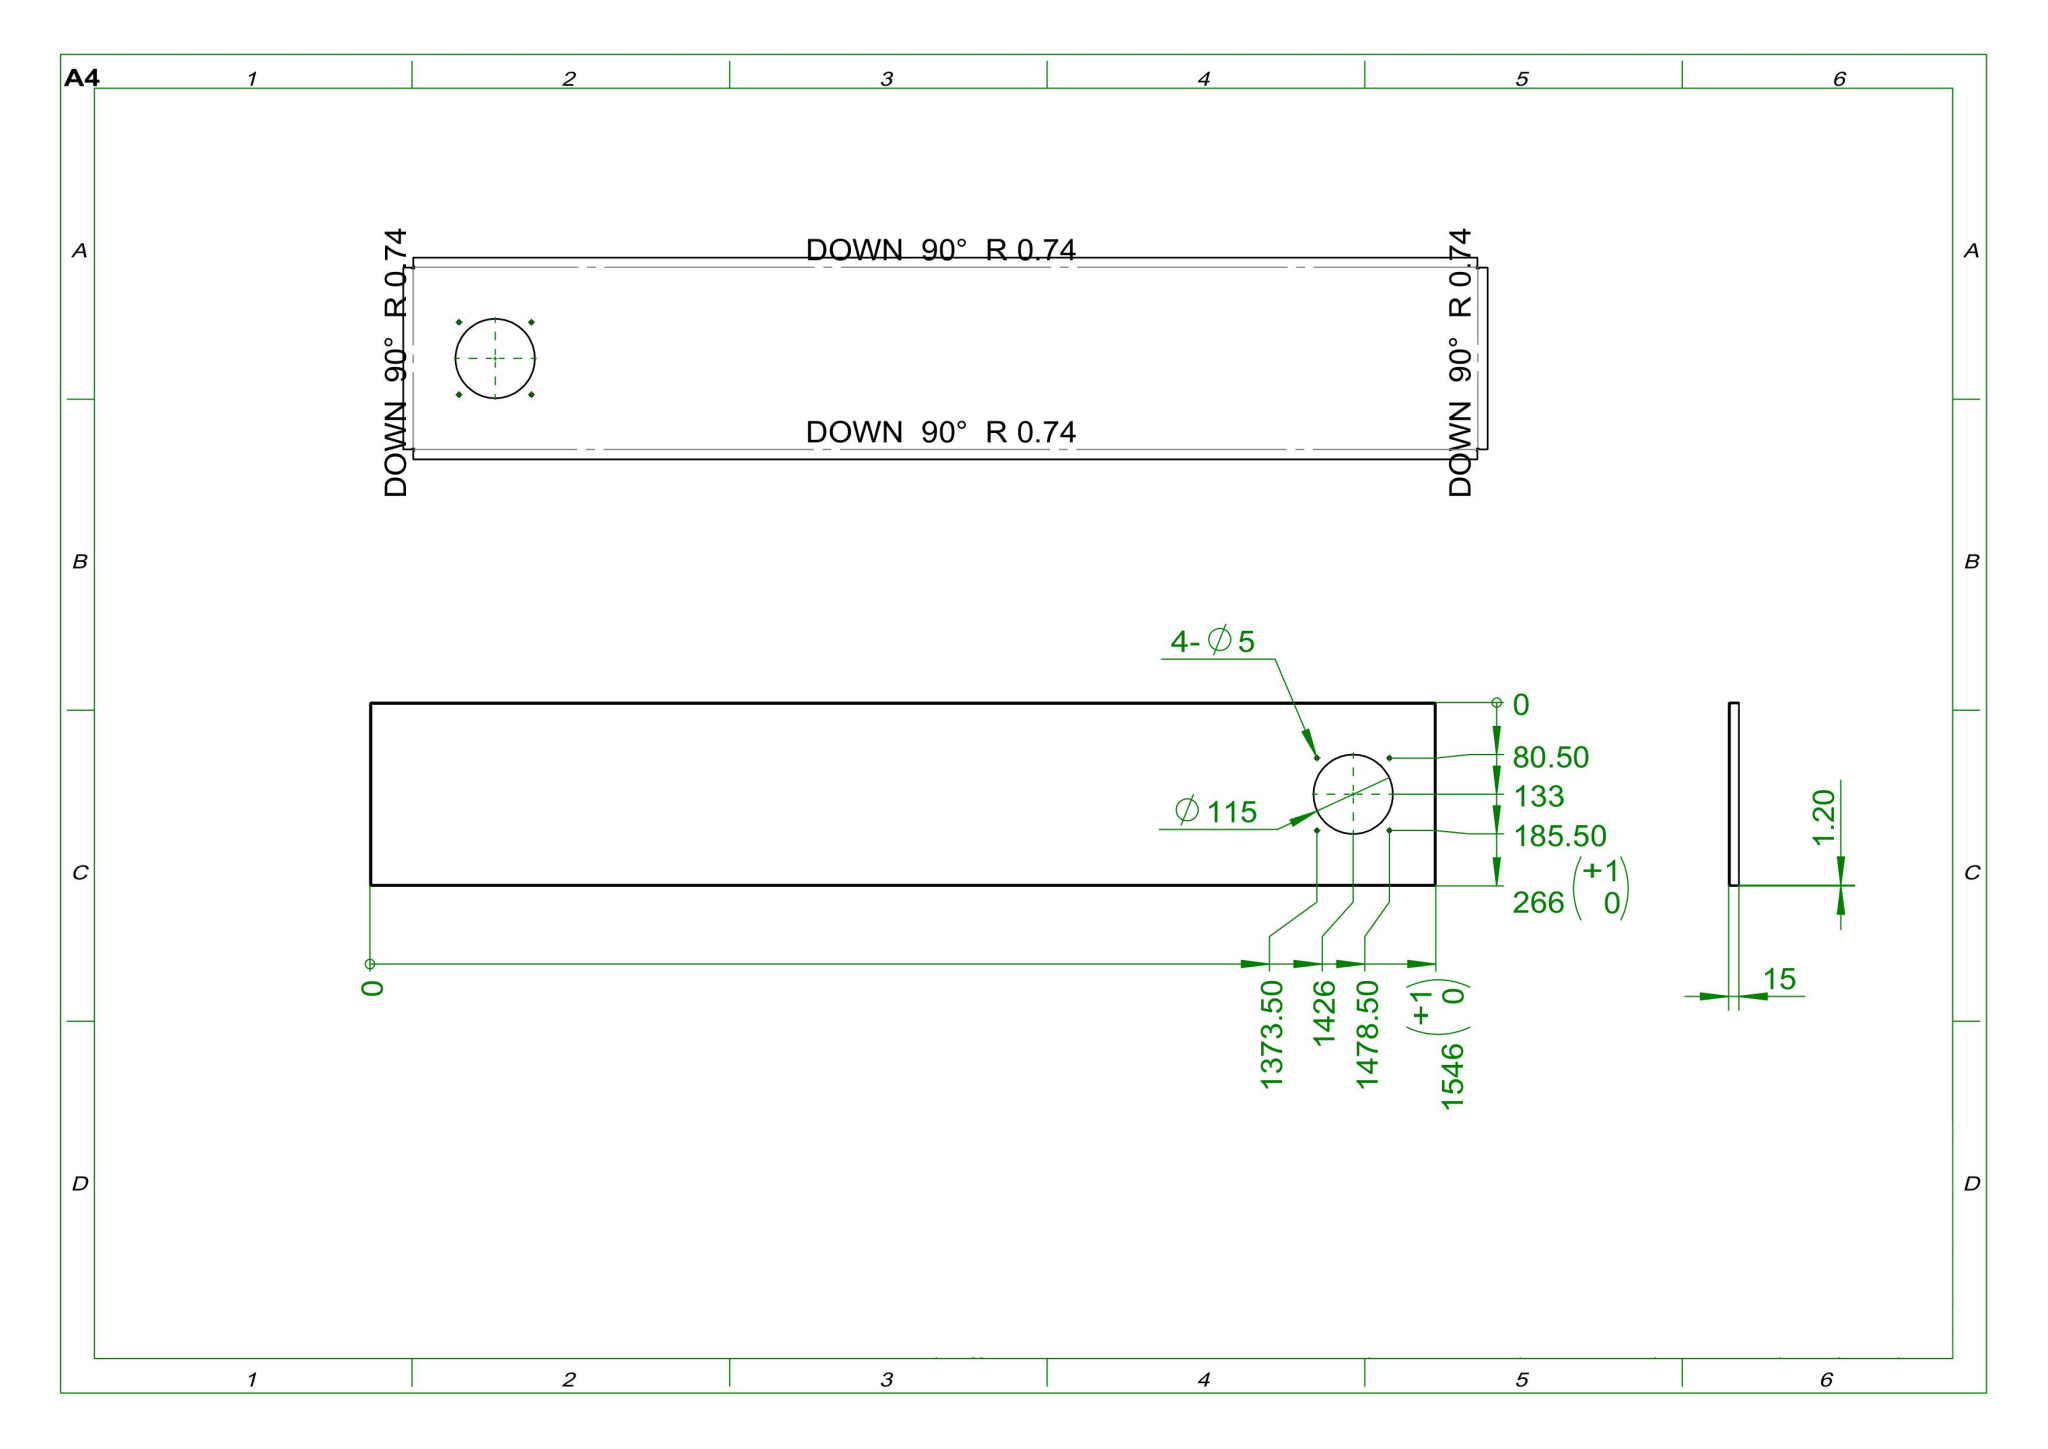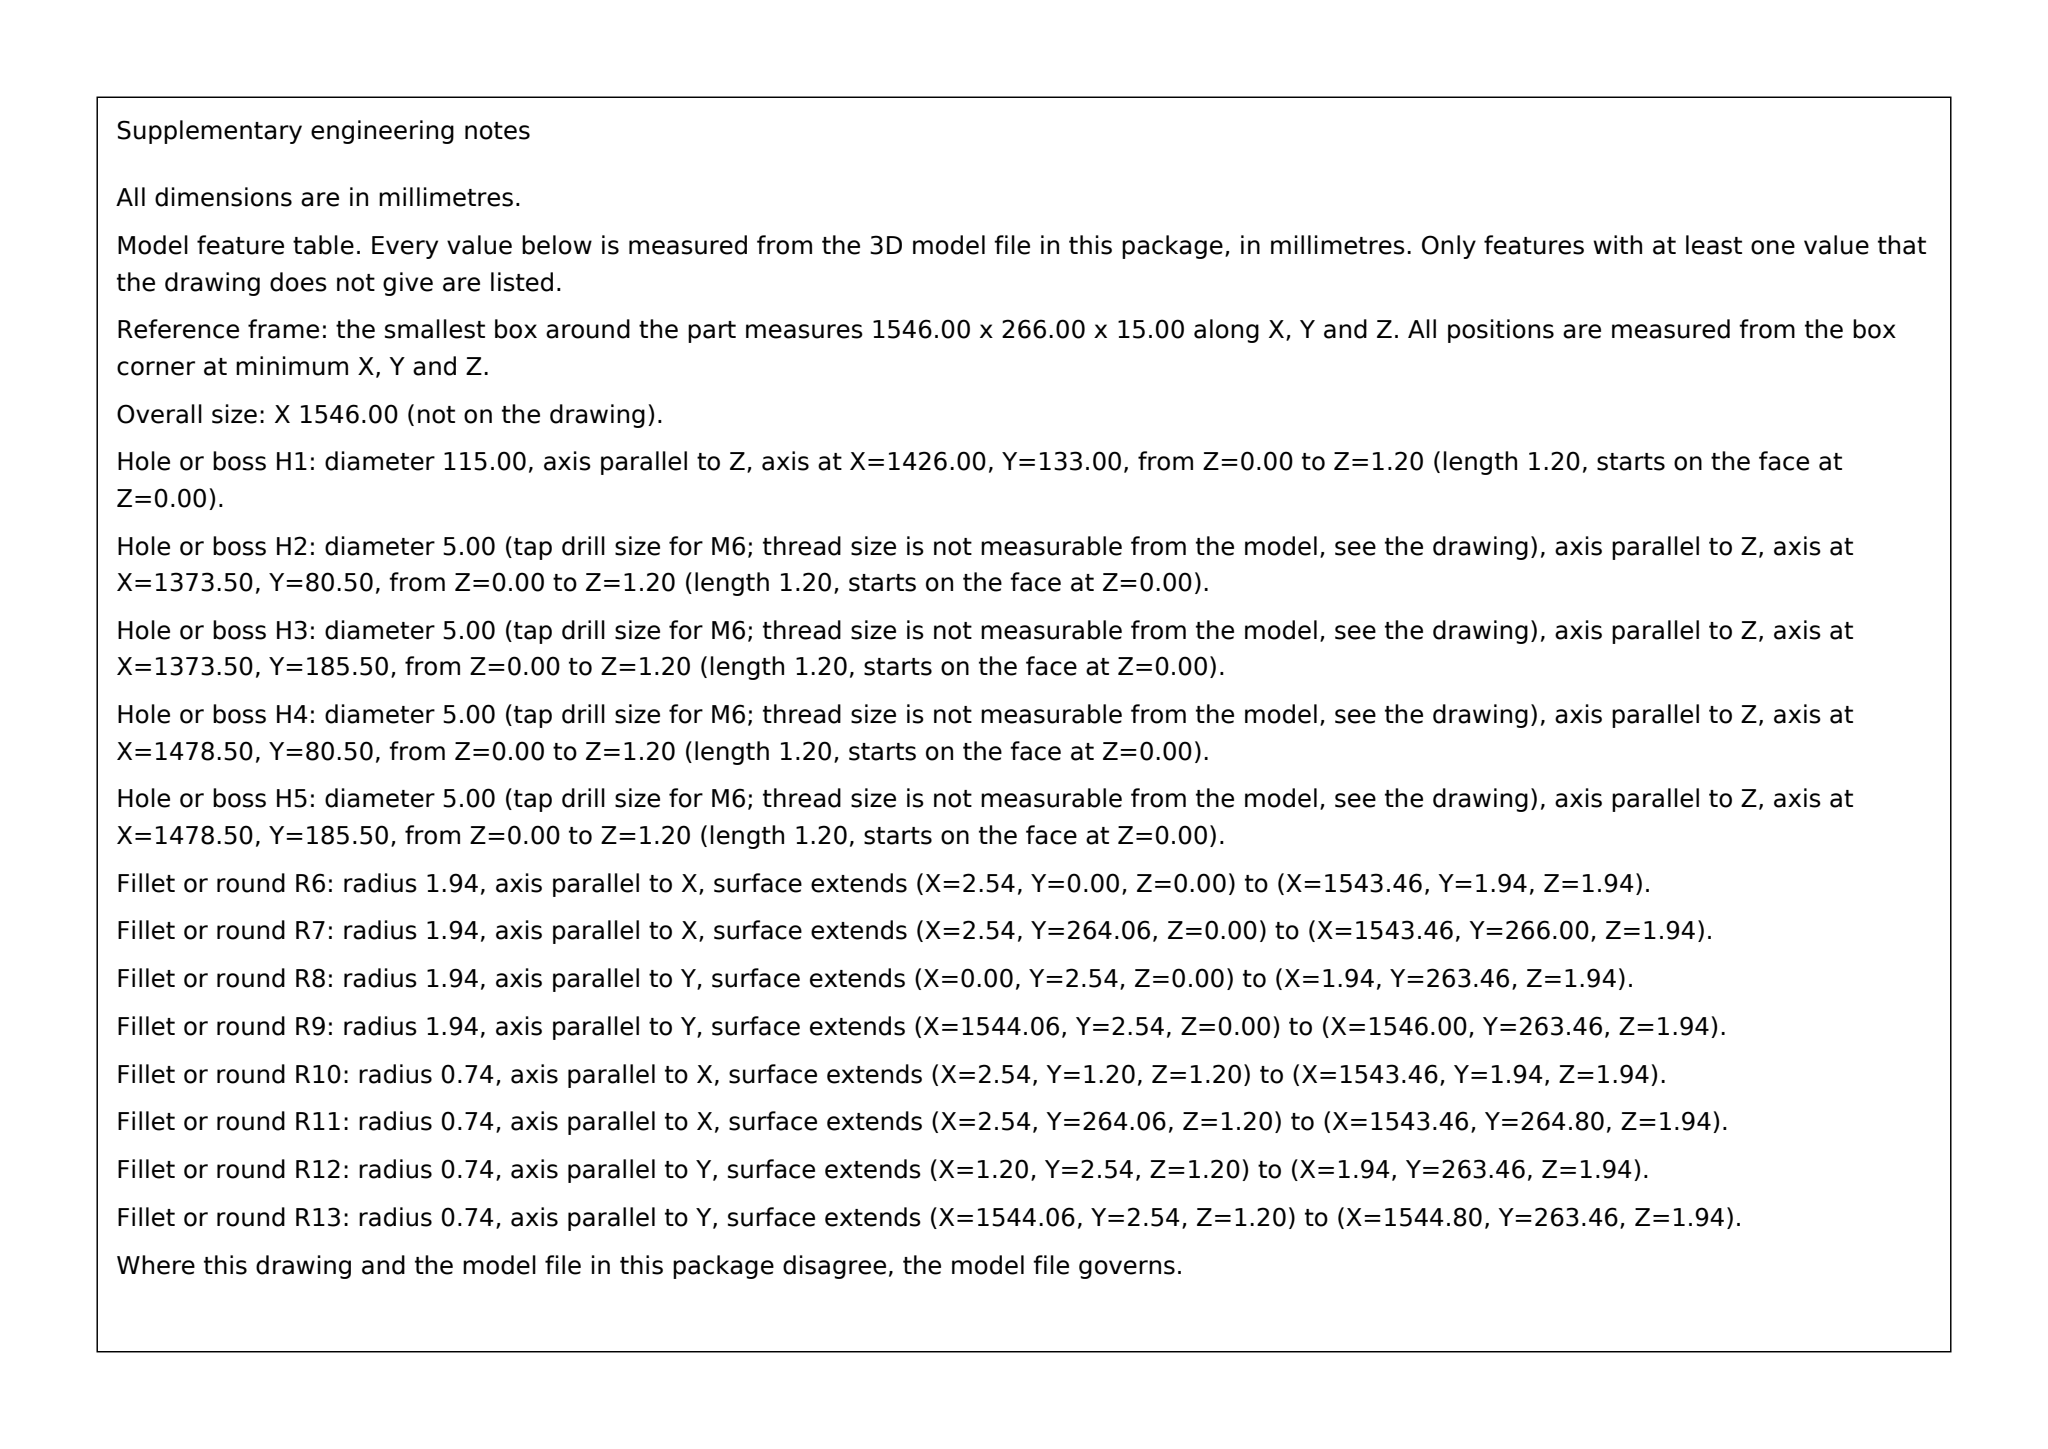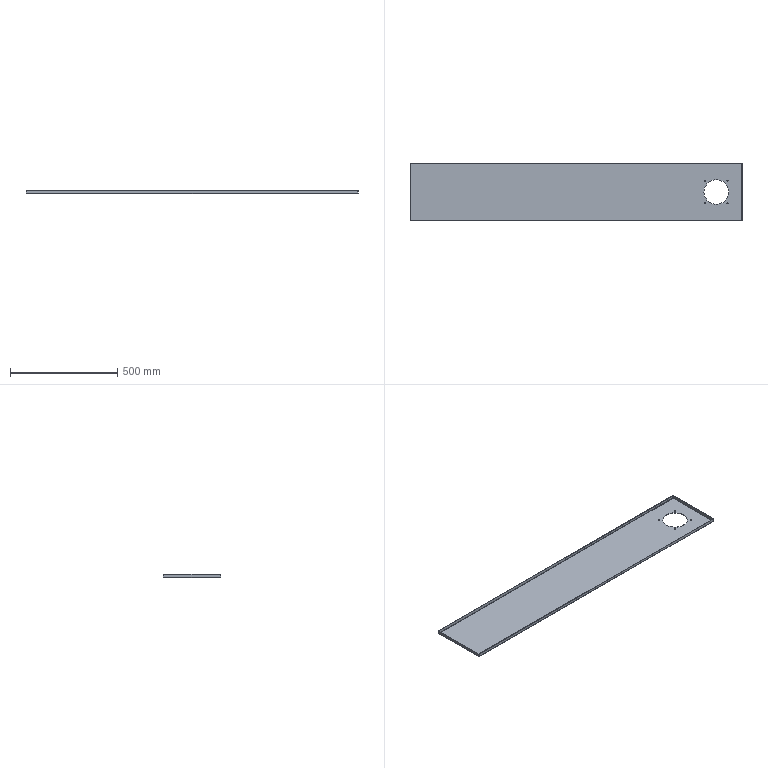Part | SolidWorks | mm | 1 solid | 72 faces | box 1546 x 266 x 15 mm | volume 538242 mm3 | plane 54 | cylinder 18 | commonest cylinder face diameters 5 x8 3.873 x4 1.473 x4 115 x2